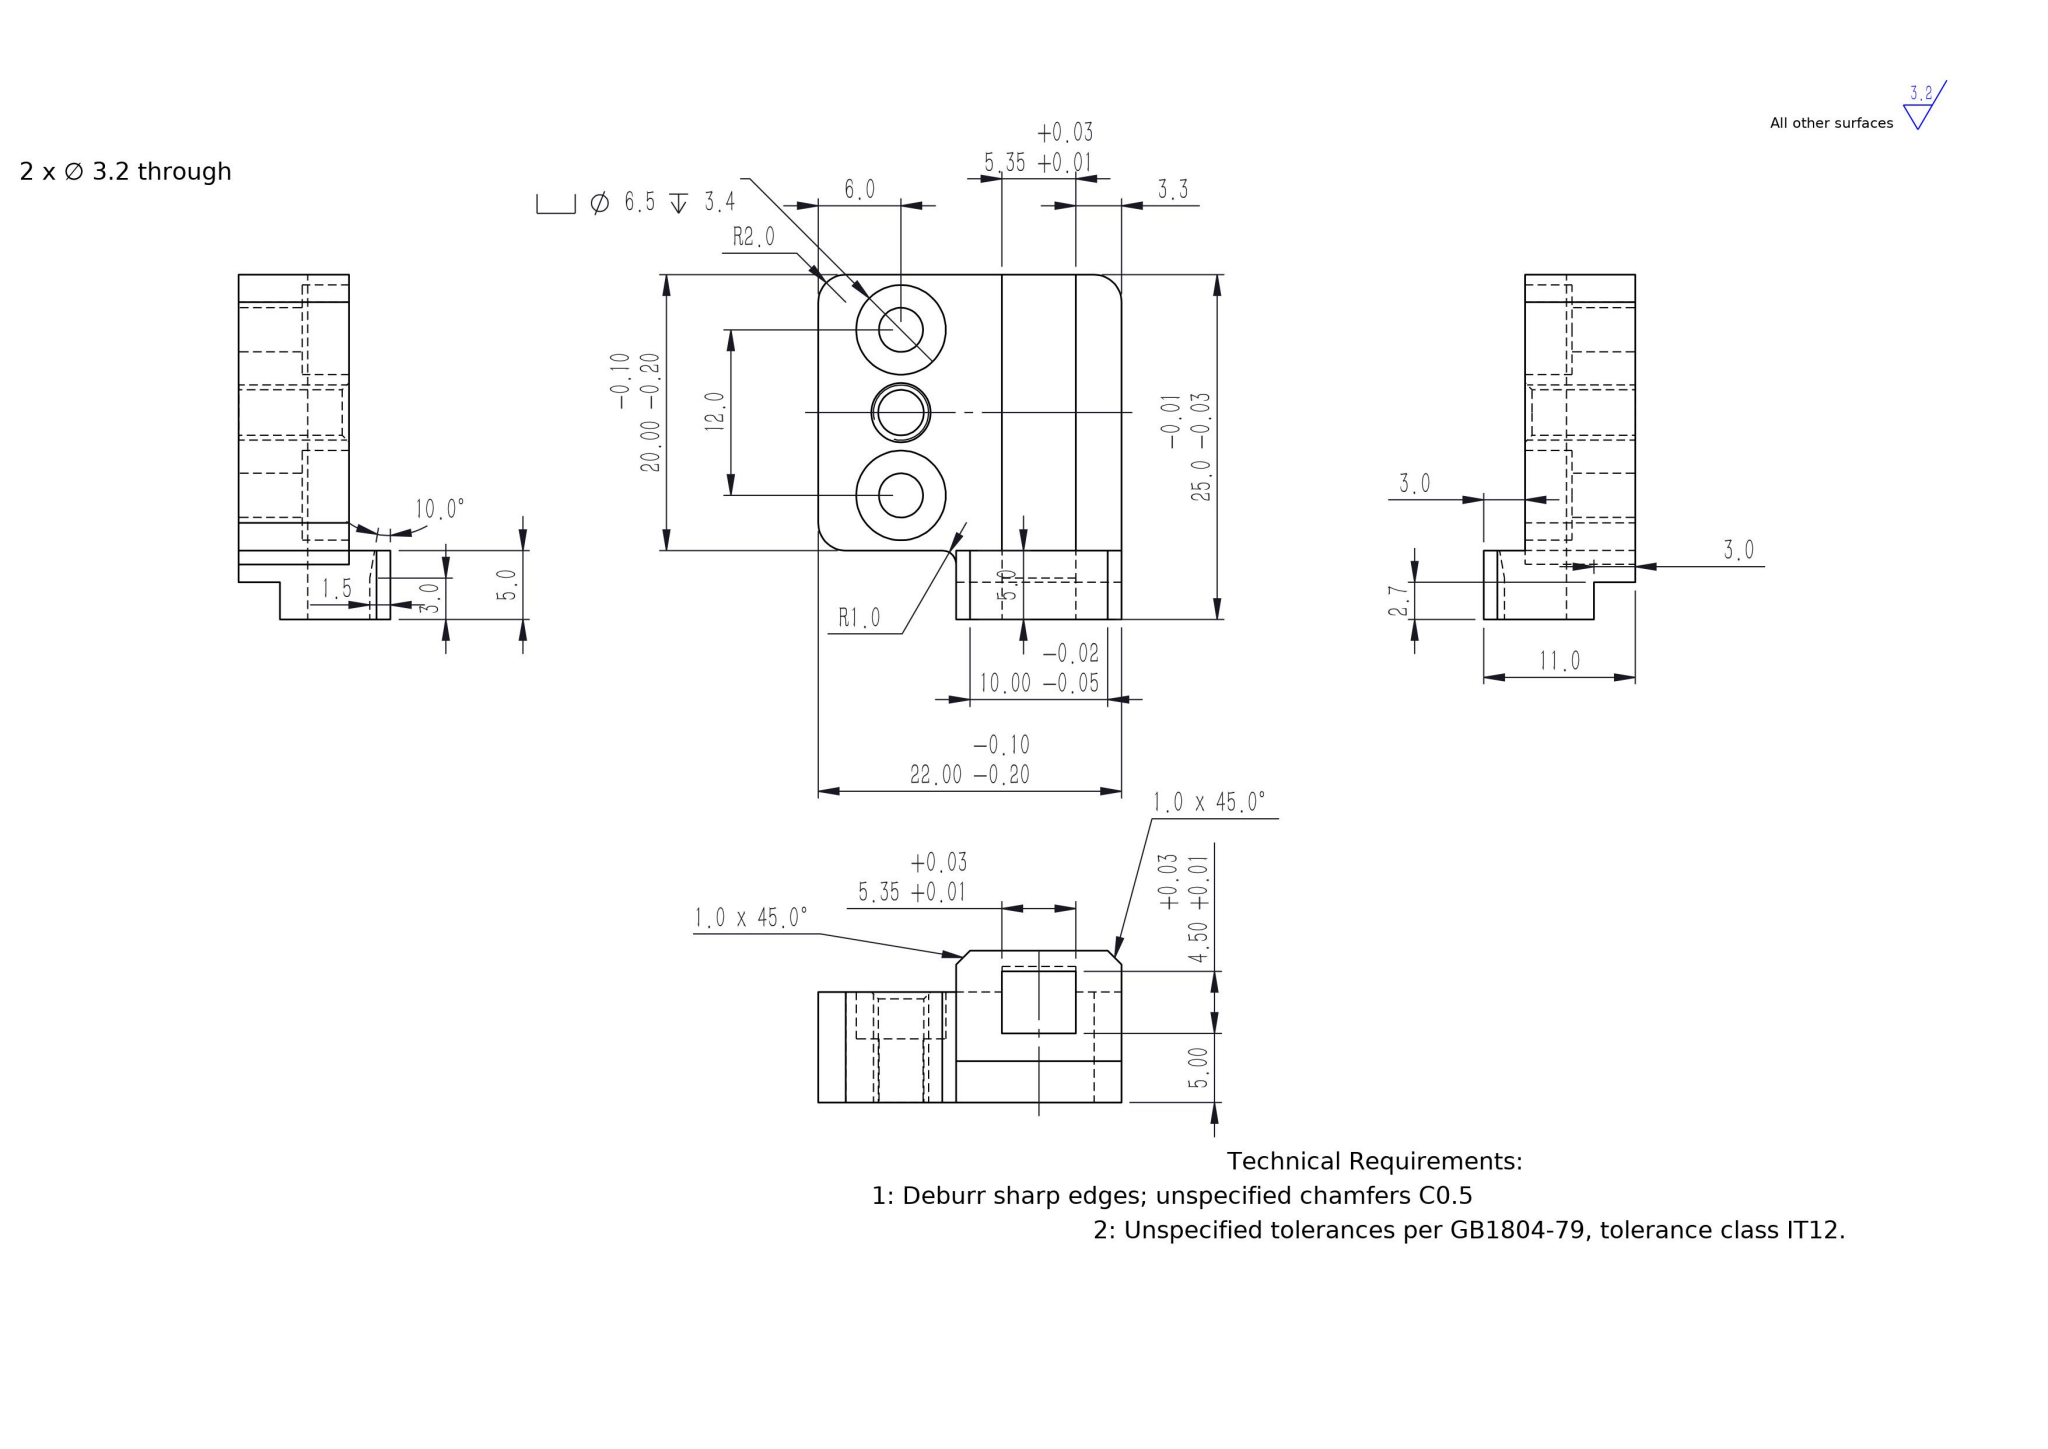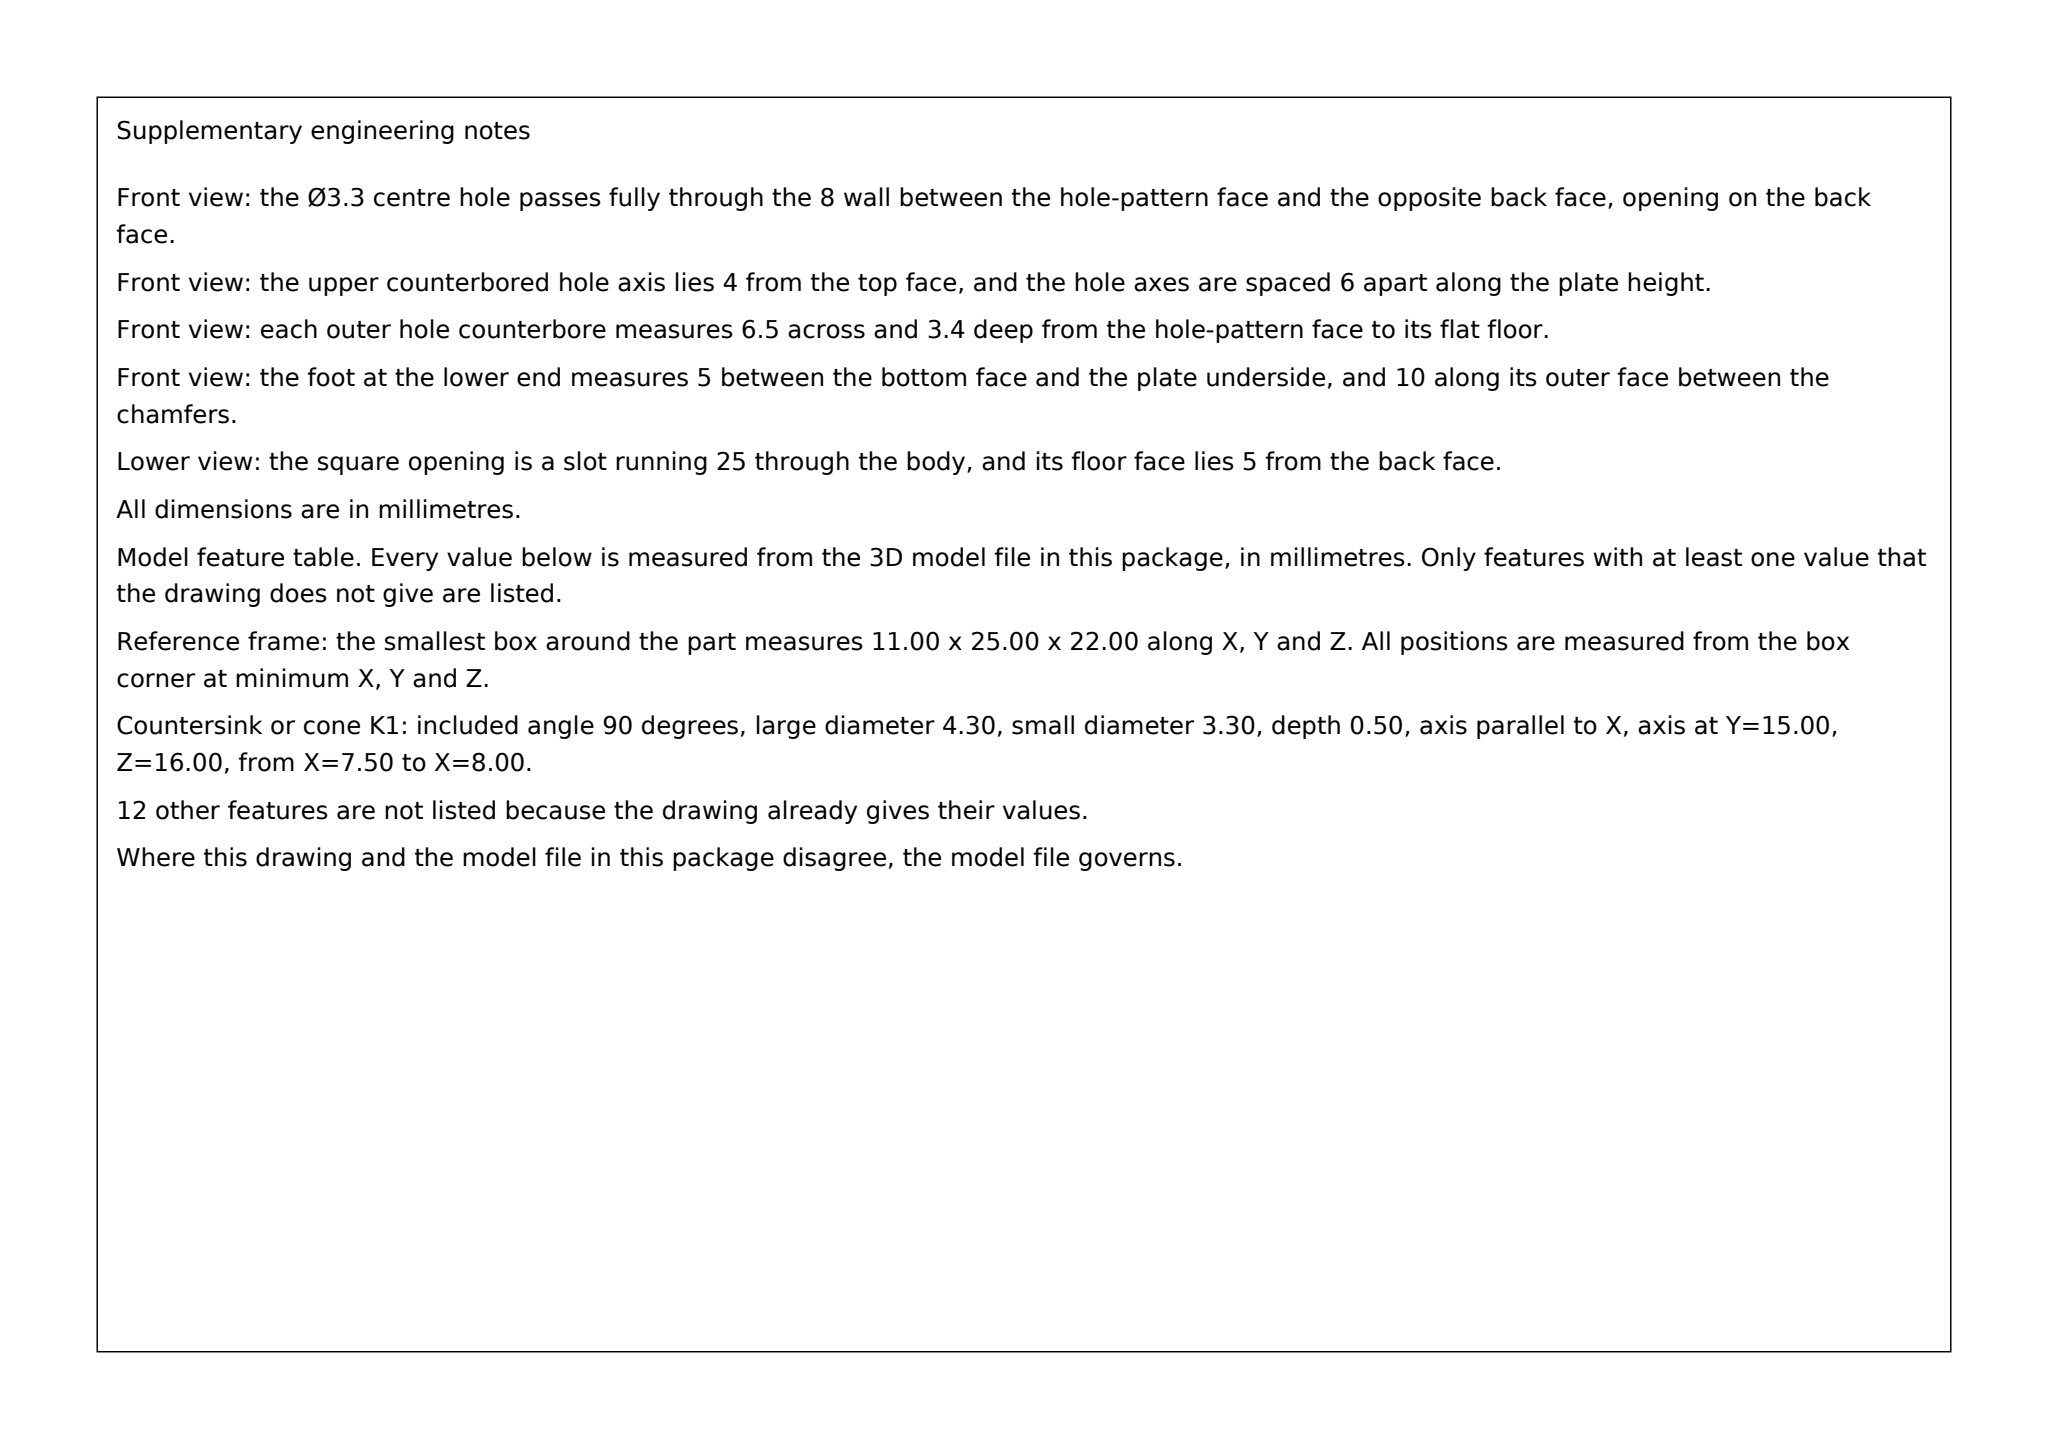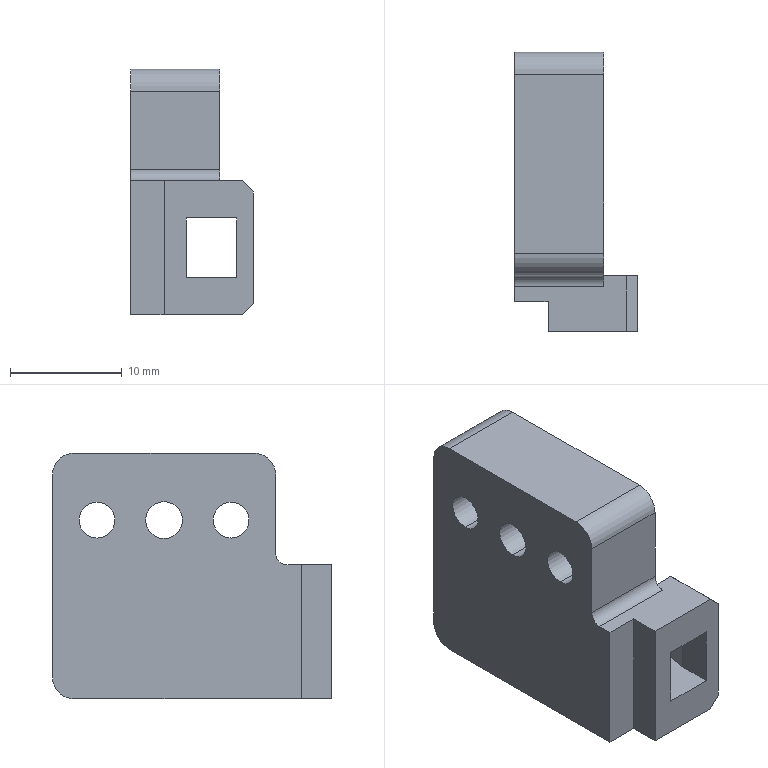Part | SolidWorks | mm | 1 solid | 38 faces | box 11 x 25 x 22 mm | volume 3246 mm3 | plane 22 | cylinder 14 | cone 2 | commonest cylinder face diameters 6.5 x4 3.2 x4 4 x3 3.3 x2 2 x1
Drawing notes:
MIDDLE HOLE: Ø3.3, ON 2X Ø3.2 HOLE CL, 6.0 FROM EA HOLE | from the solid: Cyl dia 3.3 axis x at (y=15,z=16); Ø3.2 holes at y=9 and y=21, same z=16 -> 6.0 spacing, on same vertical CL
Ø3.3 HOLE THRU ALL (8.0 PLATE THK) | from the solid: Ø3.3 cyl + 2 end cones span full plate x=0 to x=8.0 (faces x=0 and x=8.0)
Ø3.3 HOLE: CSK 90° TO Ø3.8, BOTH ENDS | from the solid: cones[included_angle,ref_dia]=90°, ref Ø3.3, qty 2; cyl length 7.5 in 8.0 thk -> 0.25 deep ea end -> 3.3+2(0.25)=Ø3.8
3-HOLE PATTERN CL 10.0 BELOW TOP FACE (15.0 ABOVE BOTTOM) | from the solid: Holes dia3.2/3.3 axes at y=9,15,21; bbox y 0-25, top face y=25 -> mid hole 10.0 from top
build123d program:
from build123d import *

# Parameters (mm, degrees)
SKETCH1_W                                       = 11
SKETCH1_H                                       = 25
BOSS_EXTRUDE1_DEPTH                             = 12
SKETCH2_W                                       = 12
SKETCH2_H                                       = 20
CUT_EXTRUDE1_DEPTH                              = 3
SKETCH3_W                                       = 4.5
SKETCH3_H                                       = 5.35
CUT_EXTRUDE2_DEPTH                              = 29.271
SKETCH4_W                                       = 12
SKETCH4_H                                       = 2.7
CUT_EXTRUDE3_DEPTH                              = 3
CHAMFER2_SIZE                                   = 2
CHAMFER2_SIZE2                                  = 0.3527
SKETCH7_W                                       = 8
SKETCH7_H                                       = 20
BOSS_EXTRUDE2_DEPTH                             = 10
M3_HEX_SOCKET_HEAD_CAP_SCREW_CBORE1_D           = 3.2
M3_HEX_SOCKET_HEAD_CAP_SCREW_CBORE1_CBORE_D     = 6.5
M3_HEX_SOCKET_HEAD_CAP_SCREW_CBORE1_CBORE_DEPTH = 3.4
FILLET1_R                                       = 2
M4_TAPPED_HOLE1_D                               = 3.3
M4_TAPPED_HOLE1_DEPTH                           = 11.5
M4_TAPPED_HOLE1_TIP                             = 0.9914
FILLET2_R                                       = 1
CHAMFER3_SIZE                                   = 1
CHAMFER4_SIZE                                   = 0.5


with BuildPart() as part:
    # Sketch1 → Boss-Extrude1 (new body)
    with BuildSketch(Plane.XY):
        Rectangle(SKETCH1_W, SKETCH1_H)
    extrude(amount=BOSS_EXTRUDE1_DEPTH)

    # Sketch2 → Cut-Extrude1 (cut)
    with BuildSketch(Plane(origin=(5.5, 0, 0), x_dir=(0, 0, -1), z_dir=(1, 0, 0))):
        with Locations((-6, 2.5)):
            Rectangle(SKETCH2_W, SKETCH2_H)
    extrude(amount=-CUT_EXTRUDE1_DEPTH, mode=Mode.SUBTRACT)

    # Sketch3 → Cut-Extrude2 (cut, through all)
    with BuildSketch(Plane(origin=(0, 12.5, 0), x_dir=(1, 0, 0), z_dir=(0, 1, 0))):
        with Locations((1.75, -6)):
            Rectangle(SKETCH3_W, SKETCH3_H)
    extrude(amount=-CUT_EXTRUDE2_DEPTH, mode=Mode.SUBTRACT)

    # Sketch4 → Cut-Extrude3 (cut)
    with BuildSketch(Plane.ZY.offset(5.5)):
        with Locations((6, -11.15)):
            Rectangle(SKETCH4_W, SKETCH4_H)
    extrude(amount=-CUT_EXTRUDE3_DEPTH, mode=Mode.SUBTRACT)

    # Chamfer2
    chamfer2_edges = [part.edges().sort_by_distance(p)[0] for p in [
        (4, -7.5, 6),
    ]]
    chamfer2_side = [part.faces().sort_by_distance(p)[0] for p in [
        (4, -10, 6),
    ]]
    chamfer(chamfer2_edges, length=CHAMFER2_SIZE, length2=CHAMFER2_SIZE2, reference=chamfer2_side[0])

    # Sketch7 → Boss-Extrude2 (add)
    with BuildSketch(Plane.XY.offset(12)):
        with Locations((-1.5, 2.5)):
            Rectangle(SKETCH7_W, SKETCH7_H)
    extrude(amount=BOSS_EXTRUDE2_DEPTH)

    # M3 Hex Socket Head Cap Screw CBORE1 (through all)
    with Locations(Plane(origin=(2.5, 0, 0), x_dir=(0, 0, -1), z_dir=(1, 0, 0))):
        with Locations((-16, 8.5), (-16, -3.5)):
            CounterBoreHole(M3_HEX_SOCKET_HEAD_CAP_SCREW_CBORE1_D / 2, M3_HEX_SOCKET_HEAD_CAP_SCREW_CBORE1_CBORE_D / 2, M3_HEX_SOCKET_HEAD_CAP_SCREW_CBORE1_CBORE_DEPTH)

    # Fillet1
    fillet1_edges = [part.edges().sort_by_distance(p)[0] for p in [
        (-1.5, 12.5, 22),
        (-1.5, 12.5, 0),
        (-1.5, -7.5, 22),
    ]]
    fillet(fillet1_edges, radius=FILLET1_R)

    # M4 Tapped Hole1
    with Locations(Plane(origin=(2.5, 0, 0), x_dir=(0, 0, -1), z_dir=(1, 0, 0))):
        with Locations((-16, 2.5)):
            Hole(M4_TAPPED_HOLE1_D / 2, depth=M4_TAPPED_HOLE1_DEPTH)
            with Locations((0, 0, -(M4_TAPPED_HOLE1_DEPTH + M4_TAPPED_HOLE1_TIP / 2))):  # 118° drill point
                Cone(0, M4_TAPPED_HOLE1_D / 2, M4_TAPPED_HOLE1_TIP, mode=Mode.SUBTRACT)

    # Fillet2
    fillet2_edges = [part.edges().sort_by_distance(p)[0] for p in [
        (-1.5, -7.5, 12),
    ]]
    fillet(fillet2_edges, radius=FILLET2_R)

    # Chamfer3
    chamfer3_edges = [part.edges().sort_by_distance(p)[0] for p in [
        (5.5, -10, 12),
        (5.5, -10, 0),
    ]]
    chamfer(chamfer3_edges, length=CHAMFER3_SIZE)

    # Chamfer4
    chamfer4_edges = [part.edges().sort_by_distance(p)[0] for p in [
        (2.5, 2.5, 14.35),
    ]]
    chamfer(chamfer4_edges, length=CHAMFER4_SIZE)


solid = part.part